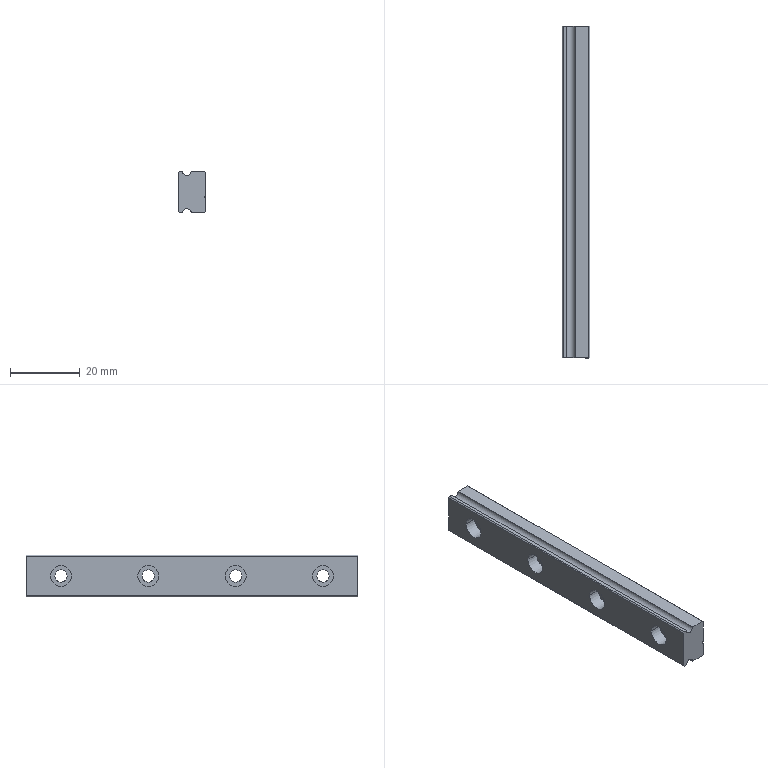Component | SolidWorks | ElectricalTestFailureExclusionLinearGuideMGN12C1R95Z0M-1_MGN12C-ElectricalTestFailureExclusionGuideRail-1 | 1 solid | 37 faces | box 8 x 95 x 12 mm | volume 8055 mm3 | cylinder 20 | plane 17 | commonest cylinder face diameters 6 x8 3.5 x8 2.5 x3 0.6 x1